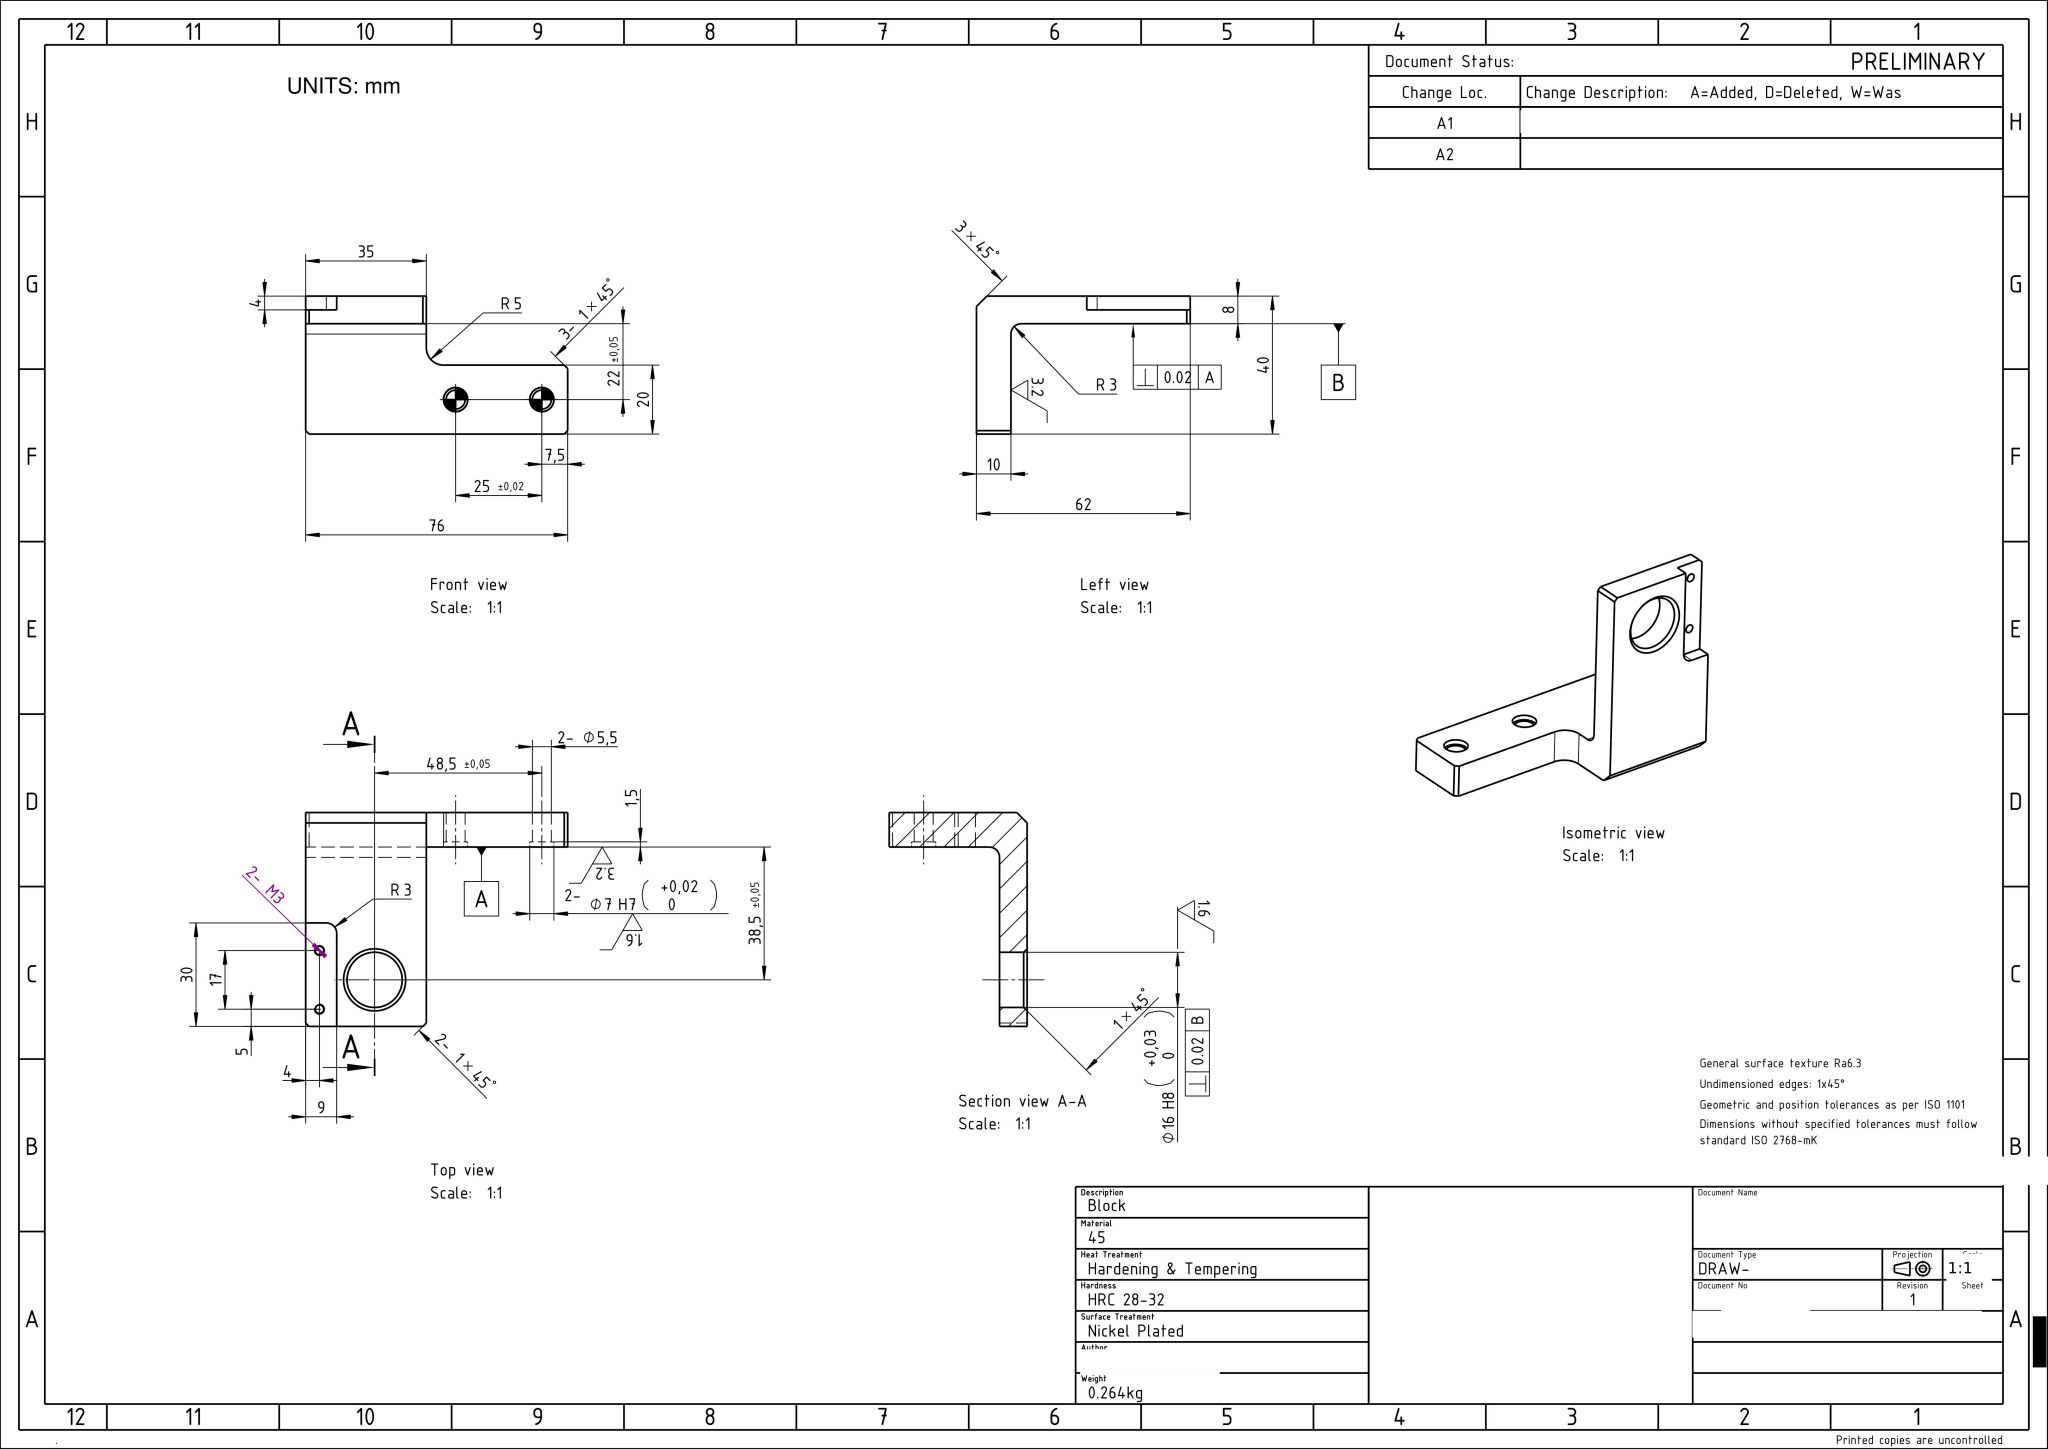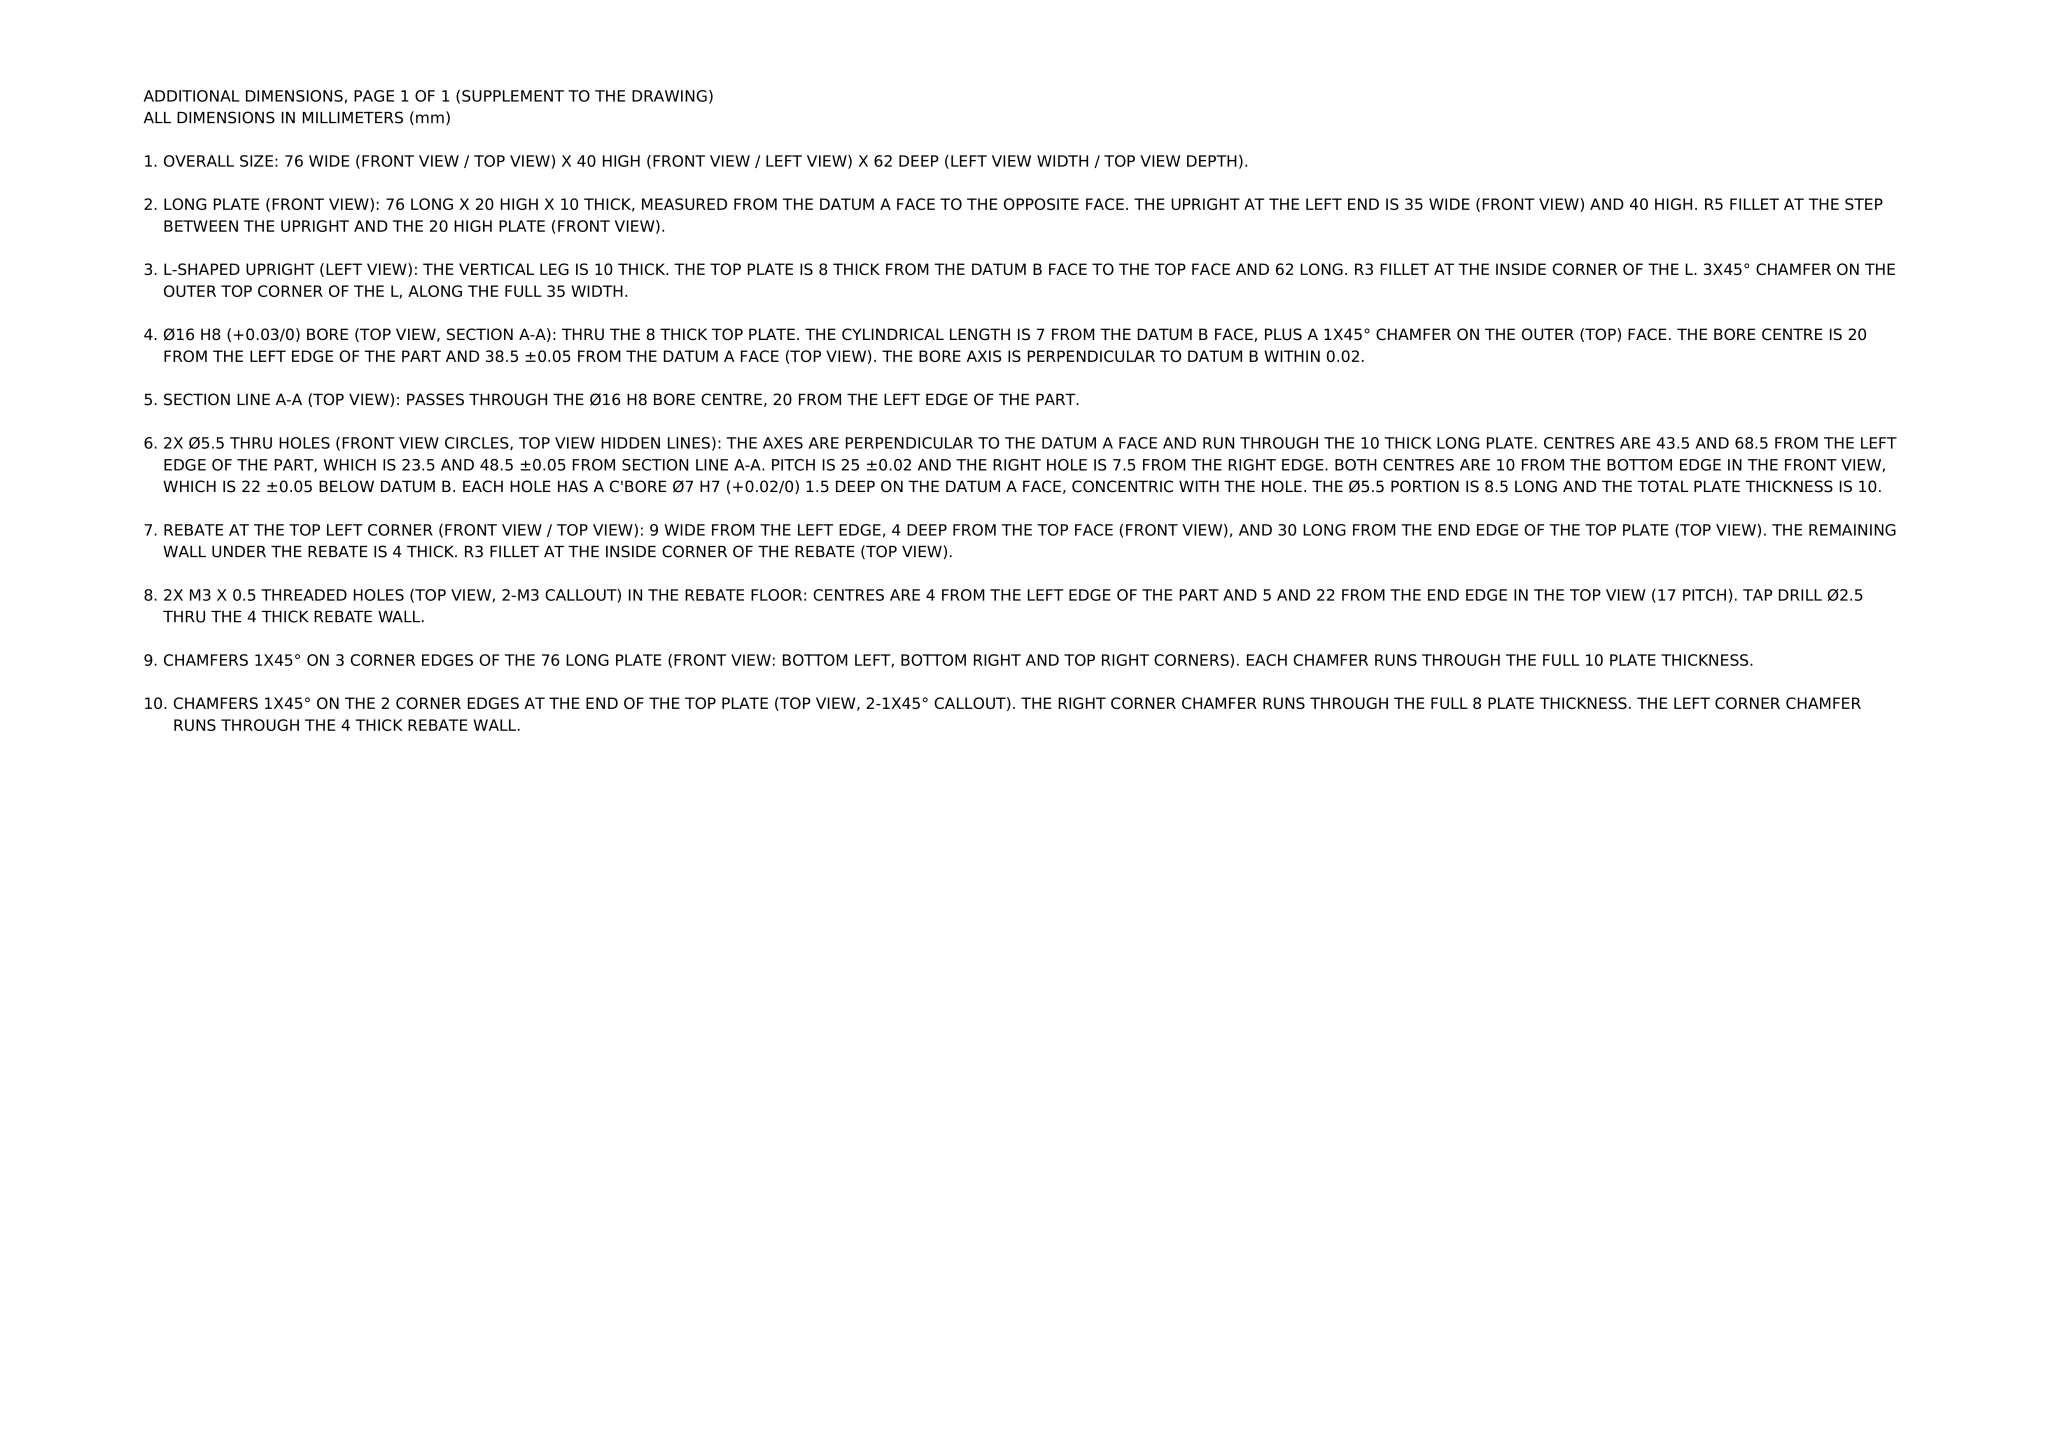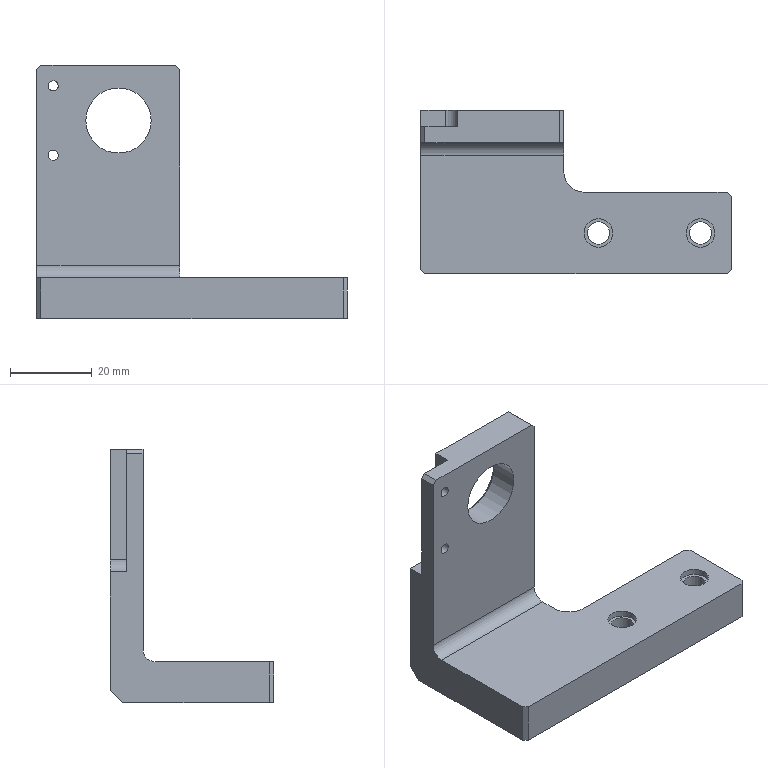Part | NX | mm | 1 solid | 32 faces | box 76 x 40 x 62 mm | volume 33437 mm3 | plane 21 | cylinder 10 | cone 1 | commonest cylinder face diameters 6 x2 5.5 x2 7 x2 2.5 x2 10 x1 16 x1